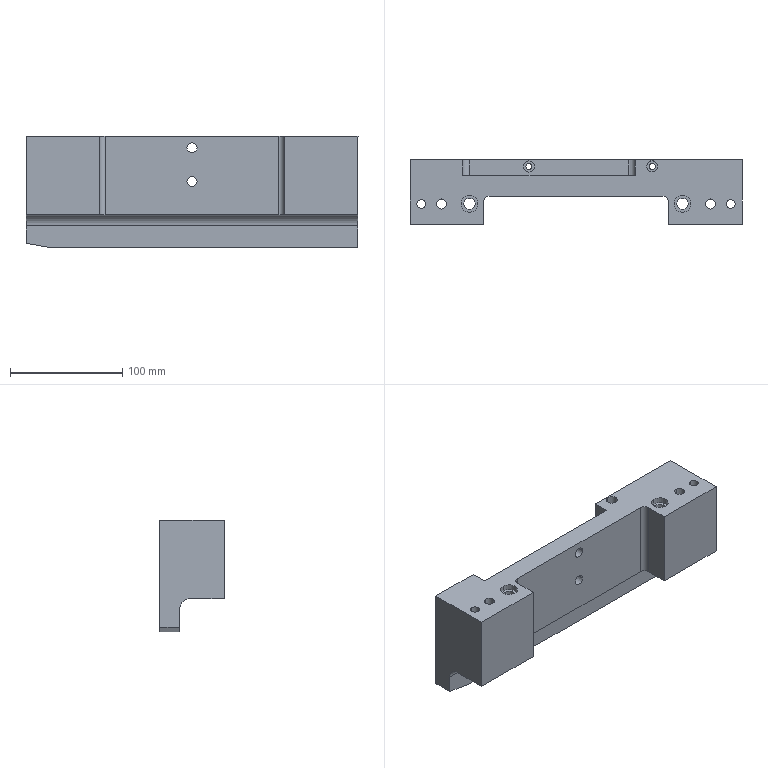Component | SolidWorks | 2SZT-2-002-2-1 | 1 solid | 84 faces | box 296 x 57.5 x 99.56 mm | volume 890252 mm3 | cylinder 49 | plane 31 | cone 4 | commonest cylinder face diameters 15 x12 9 x8 10 x6 4.01 x4 5.5 x4 8.01 x4 21 x4 10.02 x4
build123d program:
from build123d import *

# Parameters (mm, degrees)
SKETCH22_W                                           = 296
SKETCH22_H                                           = 22.5
BOSS_EXTRUDE5_DEPTH                                  = 109.55
SKETCH23_W                                           = 368.542
SKETCH23_H                                           = 48.28
CUT_EXTRUDE1_DEPTH                                   = 10
CHAMFER2_SIZE                                        = 24.5
CHAMFER2_SIZE2                                       = 1.284
SKETCH28_W                                           = 296
SKETCH28_H                                           = 70
BOSS_EXTRUDE6_DEPTH                                  = 18
SKETCH35_W                                           = 82
SKETCH35_H                                           = 70
BOSS_EXTRUDE7_DEPTH                                  = 60
SKETCH39_W                                           = 2.31
SKETCH39_H                                           = 0.5
CUT_EXTRUDE4_DEPTH                                   = 332.236
SKETCH40_R                                           = 5.01
CUT_EXTRUDE5_DEPTH                                   = 321.338
SKETCH41_R                                           = 7.5
CUT_EXTRUDE6_DEPTH                                   = 5.2
SKETCH42_R                                           = 10.5
CUT_EXTRUDE7_DEPTH                                   = 10
SKETCH43_W                                           = 60
SKETCH43_H                                           = 70
BOSS_EXTRUDE8_DEPTH                                  = 3
CUT_EXTRUDE8_START                                   = -70
SKETCH44_W                                           = 296
SKETCH44_H                                           = 42
CUT_EXTRUDE8_DEPTH                                   = 70
M8_HEX_SOCKET_HEAD_CAP_SCREW_CBORE1_D                = 9
M8_HEX_SOCKET_HEAD_CAP_SCREW_CBORE1_CBORE_D          = 15
M8_HEX_SOCKET_HEAD_CAP_SCREW_CBORE1_CBORE_DEPTH      = 25
SKETCH49_R                                           = 4.005
CUT_EXTRUDE9_DEPTH                                   = 310.739
CHAMFER4_SIZE                                        = 3
CHAMFER4_SIZE2                                       = 20
CUT_EXTRUDE11_DEPTH                                  = 70
SKETCH54_W                                           = 760.118
SKETCH54_H                                           = 551.098
CUT_EXTRUDE13_DEPTH                                  = 9.5
CHAMFER3_SIZE                                        = 4
CHAMFER3_SIZE2                                       = 22.685
CUT_EXTRUDE14_REACH                                  = 319.724
SKETCH55_W                                           = 358.749
SKETCH55_H                                           = 98.379
FILLET3_R                                            = 10
SKETCH56_W                                           = 250
SKETCH56_H                                           = 30.92
CUT_EXTRUDE15_DEPTH                                  = 4
M5_HEX_SOCKET_HEAD_CAP_SCREW_CBORE1_D                = 5.5
M5_HEX_SOCKET_HEAD_CAP_SCREW_CBORE1_CBORE_D          = 10
M5_HEX_SOCKET_HEAD_CAP_SCREW_CBORE1_CBORE_DEPTH      = 60
F_4_0_4_DIAMETER_HOLE1_D                             = 4.01
F_4_0_4_DIAMETER_HOLE1_DEPTH                         = 20
F_4_0_4_DIAMETER_HOLE1_TIP                           = 1.205
SKETCH67_W                                           = 154
SKETCH67_H                                           = 61.336
CUT_EXTRUDE16_DEPTH                                  = 15
FILLET4_R                                            = 6
SKETCH68_W                                           = 783.965
SKETCH68_H                                           = 336.436
CUT_EXTRUDE17_DEPTH                                  = 1
HOLE_SIZE_ACCORDING_TO_THE_TYPE_OF_HEXAG_D           = 9
HOLE_SIZE_ACCORDING_TO_THE_TYPE_OF_HEXAG_CBORE_D     = 15
HOLE_SIZE_ACCORDING_TO_THE_TYPE_OF_HEXAG_CBORE_DEPTH = 8.5


with BuildPart() as part:
    # Sketch22 → Boss-Extrude5 (new body)
    with BuildSketch(Plane(origin=(0, 0, 0), x_dir=(1, 0, 0), z_dir=(0, 1, 0))):
        with Locations((-148, 11.25)):
            Rectangle(SKETCH22_W, SKETCH22_H)
    extrude(amount=BOSS_EXTRUDE5_DEPTH)

    # Sketch23 → Cut-Extrude1 (cut)
    with BuildSketch(Plane(origin=(0, 109.55, 0), x_dir=(1, 0, 0), z_dir=(0, 1, 0))):
        with Locations((-166.239, -3.95)):
            Rectangle(SKETCH23_W, SKETCH23_H)
    extrude(amount=-CUT_EXTRUDE1_DEPTH, mode=Mode.SUBTRACT)

    # Chamfer2
    chamfer2_edges = [part.edges().sort_by_distance(p)[0] for p in [
        (-296, 104.55, -20.19),
    ]]
    chamfer2_side = [part.faces().sort_by_distance(p)[0] for p in [
        (-148, 104.55, -20.19),
    ]]
    chamfer(chamfer2_edges, length=CHAMFER2_SIZE, length2=CHAMFER2_SIZE2, reference=chamfer2_side[0])

    # Sketch28 → Boss-Extrude6 (add)
    with BuildSketch(Plane(origin=(0, 0, -22.5), x_dir=(-1, 0, 0), z_dir=(0, 0, -1))):
        with Locations((148, 35)):
            Rectangle(SKETCH28_W, SKETCH28_H)
    extrude(amount=BOSS_EXTRUDE6_DEPTH)

    # Sketch35 → Boss-Extrude7 (add)
    with BuildSketch(Plane(origin=(0, 0, -40.5), x_dir=(-1, 0, 0), z_dir=(0, 0, -1))):
        with Locations((41, 35)):
            Rectangle(SKETCH35_W, SKETCH35_H)
        with Locations((255, 35)):
            Rectangle(SKETCH35_W, SKETCH35_H)
    extrude(amount=BOSS_EXTRUDE7_DEPTH)

    # Sketch39 → Cut-Extrude4 (cut, through all)
    with BuildSketch(Plane.ZY.offset(296)):
        with Locations((-21.345, 109.3)):
            Rectangle(SKETCH39_W, SKETCH39_H)
    extrude(amount=-CUT_EXTRUDE4_DEPTH, mode=Mode.SUBTRACT)

    # Sketch40 → Cut-Extrude5 (cut, through all)
    with BuildSketch(Plane(origin=(0, 70, 0), x_dir=(1, 0, 0), z_dir=(0, 1, 0))):
        with Locations(Location((-53, 40.27, 0), (0, 0, 270))):
            Circle(SKETCH40_R)
        with Locations(Location((-243, 40.27, 0), (0, 0, 270))):
            Circle(SKETCH40_R)
    extrude(amount=-CUT_EXTRUDE5_DEPTH, mode=Mode.SUBTRACT)

    # Sketch41 → Cut-Extrude6 (cut)
    with BuildSketch(Plane.XZ):
        with Locations(Location((-243, -40.27, 0), (0, 0, 270))):
            Circle(SKETCH41_R)
        with Locations(Location((-53, -40.27, 0), (0, 0, 270))):
            Circle(SKETCH41_R)
    extrude(amount=-CUT_EXTRUDE6_DEPTH, mode=Mode.SUBTRACT)

    # Sketch42 → Cut-Extrude7 (cut)
    with BuildSketch(Plane(origin=(0, 70, 0), x_dir=(1, 0, 0), z_dir=(0, 1, 0))):
        with Locations(Location((-243, 40.27, 0), (0, 0, 270))):
            Circle(SKETCH42_R)
        with Locations(Location((-53, 40.27, 0), (0, 0, 270))):
            Circle(SKETCH42_R)
    extrude(amount=-CUT_EXTRUDE7_DEPTH, mode=Mode.SUBTRACT)

    # Sketch43 → Boss-Extrude8 (add)
    with BuildSketch(Plane(origin=(-214, 0, 0), x_dir=(0, 0, -1), z_dir=(1, 0, 0))):
        with Locations((70.5, 35)):
            Rectangle(SKETCH43_W, SKETCH43_H)
    extrude(amount=BOSS_EXTRUDE8_DEPTH)

    # Sketch44 → Cut-Extrude8 (cut)
    with BuildSketch(Plane(origin=(0, 70, 0), x_dir=(1, 0, 0), z_dir=(0, 1, 0)).offset(CUT_EXTRUDE8_START)):
        with Locations((-148, 79.5)):
            Rectangle(SKETCH44_W, SKETCH44_H)
    extrude(amount=CUT_EXTRUDE8_DEPTH, mode=Mode.SUBTRACT)

    # M8 Hex Socket Head Cap Screw CBORE1 (through all)
    with Locations(Plane(origin=(0, 70, 0), x_dir=(1, 0, 0), z_dir=(0, 1, 0))):
        with Locations((-268, 40.5), (-28, 40.5)):
            CounterBoreHole(M8_HEX_SOCKET_HEAD_CAP_SCREW_CBORE1_D / 2, M8_HEX_SOCKET_HEAD_CAP_SCREW_CBORE1_CBORE_D / 2, M8_HEX_SOCKET_HEAD_CAP_SCREW_CBORE1_CBORE_DEPTH)

    # Sketch49 → Cut-Extrude9 (cut, through all)
    with BuildSketch(Plane(origin=(0, 70, 0), x_dir=(1, 0, 0), z_dir=(0, 1, 0))):
        with Locations(Location((-10, 40.5, 0), (0, 0, 270))):
            Circle(SKETCH49_R)
        with Locations(Location((-286, 40.5, 0), (0, 0, 270))):
            Circle(SKETCH49_R)
    extrude(amount=-CUT_EXTRUDE9_DEPTH, mode=Mode.SUBTRACT)

    # Chamfer4
    chamfer4_edges = [part.edges().sort_by_distance(p)[0] for p in [
        (-296, 109.05, -21.987),
    ]]
    chamfer4_side = [part.faces().sort_by_distance(p)[0] for p in [
        (-296, 42.08, -26.726),
    ]]
    chamfer(chamfer4_edges, length=CHAMFER4_SIZE, length2=CHAMFER4_SIZE2, reference=chamfer4_side[0])

    # Sketch52 → Cut-Extrude11 (cut)
    with BuildSketch(Plane(origin=(0, 70, 0), x_dir=(1, 0, 0), z_dir=(0, 1, 0))):
        with BuildLine():
            Line((-225.5, 33.5), (-70.5, 33.5))
            ThreePointArc((-70.5, 33.5), (-66.964, 34.964), (-65.5, 38.5))
            Line((-65.5, 38.5), (-65.5, 82.998))
            Line((-65.5, 82.998), (-230.5, 82.998))
            Line((-230.5, 82.998), (-230.5, 38.5))
            ThreePointArc((-230.5, 38.5), (-229.036, 34.964), (-225.5, 33.5))
        make_face()
    extrude(amount=-CUT_EXTRUDE11_DEPTH, mode=Mode.SUBTRACT)

    # Sketch54 → Cut-Extrude13 (cut)
    with BuildSketch(Plane(origin=(0, 109.05, 0), x_dir=(1, 0, 0), z_dir=(0, 1, 0))):
        with Locations((-135.319, 22.109)):
            Rectangle(SKETCH54_W, SKETCH54_H)
    extrude(amount=-CUT_EXTRUDE13_DEPTH, mode=Mode.SUBTRACT)

    # Chamfer3
    chamfer3_edges = [part.edges().sort_by_distance(p)[0] for p in [
        (-296, 99.55, -11.25),
    ]]
    chamfer3_side = [part.faces().sort_by_distance(p)[0] for p in [
        (-296, 41.953, -26.736),
    ]]
    chamfer(chamfer3_edges, length=CHAMFER3_SIZE, length2=CHAMFER3_SIZE2, reference=chamfer3_side[0])

    # Cut-Extrude14: up to this face of the body (flat: up to its plane)
    cut_extrude14_end = Plane(part.part.faces().sort_by_distance((-148, 70, -25.482))[0])
    # Sketch55 → Cut-Extrude14 (cut, up to the picked face)
    with BuildSketch(Plane(origin=(0, 99.55, 0), x_dir=(1, 0, 0), z_dir=(0, 1, 0)), mode=Mode.PRIVATE) as cut_extrude14_sk1:
        with Locations((-137.438, 67.689)):
            Rectangle(SKETCH55_W, SKETCH55_H)
    cut_extrude14_tool1 = split(extrude(cut_extrude14_sk1.sketch, amount=-CUT_EXTRUDE14_REACH, mode=Mode.PRIVATE), bisect_by=cut_extrude14_end, keep=Keep.BOTH, mode=Mode.PRIVATE)
    add(cut_extrude14_tool1.solids().sort_by(Axis((-137.438, 99.55, -67.689), (0, -1, 0)))[0], mode=Mode.SUBTRACT)

    # Fillet3
    fillet3_edges = [part.edges().sort_by_distance(p)[0] for p in [
        (-148, 70, -18.5),
    ]]
    fillet(fillet3_edges, radius=FILLET3_R)

    # Sketch56 → Cut-Extrude15 (cut)
    with BuildSketch(Plane(origin=(0, 99.55, 0), x_dir=(1, 0, 0), z_dir=(0, 1, 0))):
        with Locations((-135, -1.27)):
            Rectangle(SKETCH56_W, SKETCH56_H)
    extrude(amount=-CUT_EXTRUDE15_DEPTH, mode=Mode.SUBTRACT)

    # M5 Hex Socket Head Cap Screw CBORE1 (through all)
    with Locations(Plane(origin=(0, 0, 0), x_dir=(-1, 0, 0), z_dir=(0, -1, 0))):
        with Locations((190, 6.94), (80, 6.94)):
            CounterBoreHole(M5_HEX_SOCKET_HEAD_CAP_SCREW_CBORE1_D / 2, M5_HEX_SOCKET_HEAD_CAP_SCREW_CBORE1_CBORE_D / 2, M5_HEX_SOCKET_HEAD_CAP_SCREW_CBORE1_CBORE_DEPTH)

    # 4.0 _4_ Diameter Hole1
    with Locations(Plane(origin=(0, 95.55, 0), x_dir=(1, 0, 0), z_dir=(0, 1, 0))):
        with Locations((-50, 6.94), (-220, 6.94)):
            Hole(F_4_0_4_DIAMETER_HOLE1_D / 2, depth=F_4_0_4_DIAMETER_HOLE1_DEPTH)
            with Locations((0, 0, -(F_4_0_4_DIAMETER_HOLE1_DEPTH + F_4_0_4_DIAMETER_HOLE1_TIP / 2))):  # 118° drill point
                Cone(0, F_4_0_4_DIAMETER_HOLE1_D / 2, F_4_0_4_DIAMETER_HOLE1_TIP, mode=Mode.SUBTRACT)

    # Sketch67 → Cut-Extrude16 (cut)
    with BuildSketch(Plane.XY):
        with Locations((-172, 19.332)):
            Rectangle(SKETCH67_W, SKETCH67_H)
    extrude(amount=-CUT_EXTRUDE16_DEPTH, mode=Mode.SUBTRACT)

    # Fillet4
    fillet4_edges = [part.edges().sort_by_distance(p)[0] for p in [
        (-95, 50, -7.5),
        (-249, 50, -7.5),
    ]]
    fillet(fillet4_edges, radius=FILLET4_R)

    # Sketch68 → Cut-Extrude17 (cut)
    with BuildSketch(Plane.XY):
        with Locations((-201.008, 12.225)):
            Rectangle(SKETCH68_W, SKETCH68_H)
    extrude(amount=-CUT_EXTRUDE17_DEPTH, mode=Mode.SUBTRACT)

    # Hole Size according to the type of hexag (through all)
    with Locations(Plane.XY.offset(-15)):
        with Locations((-148, 40.319), (-148, 10.319)):
            CounterBoreHole(HOLE_SIZE_ACCORDING_TO_THE_TYPE_OF_HEXAG_D / 2, HOLE_SIZE_ACCORDING_TO_THE_TYPE_OF_HEXAG_CBORE_D / 2, HOLE_SIZE_ACCORDING_TO_THE_TYPE_OF_HEXAG_CBORE_DEPTH)


solid = part.part

# Placed as in the assembly
solid = solid.moved(Location((1103.267, 424.655, -175.946), (-90, 0, 0)))